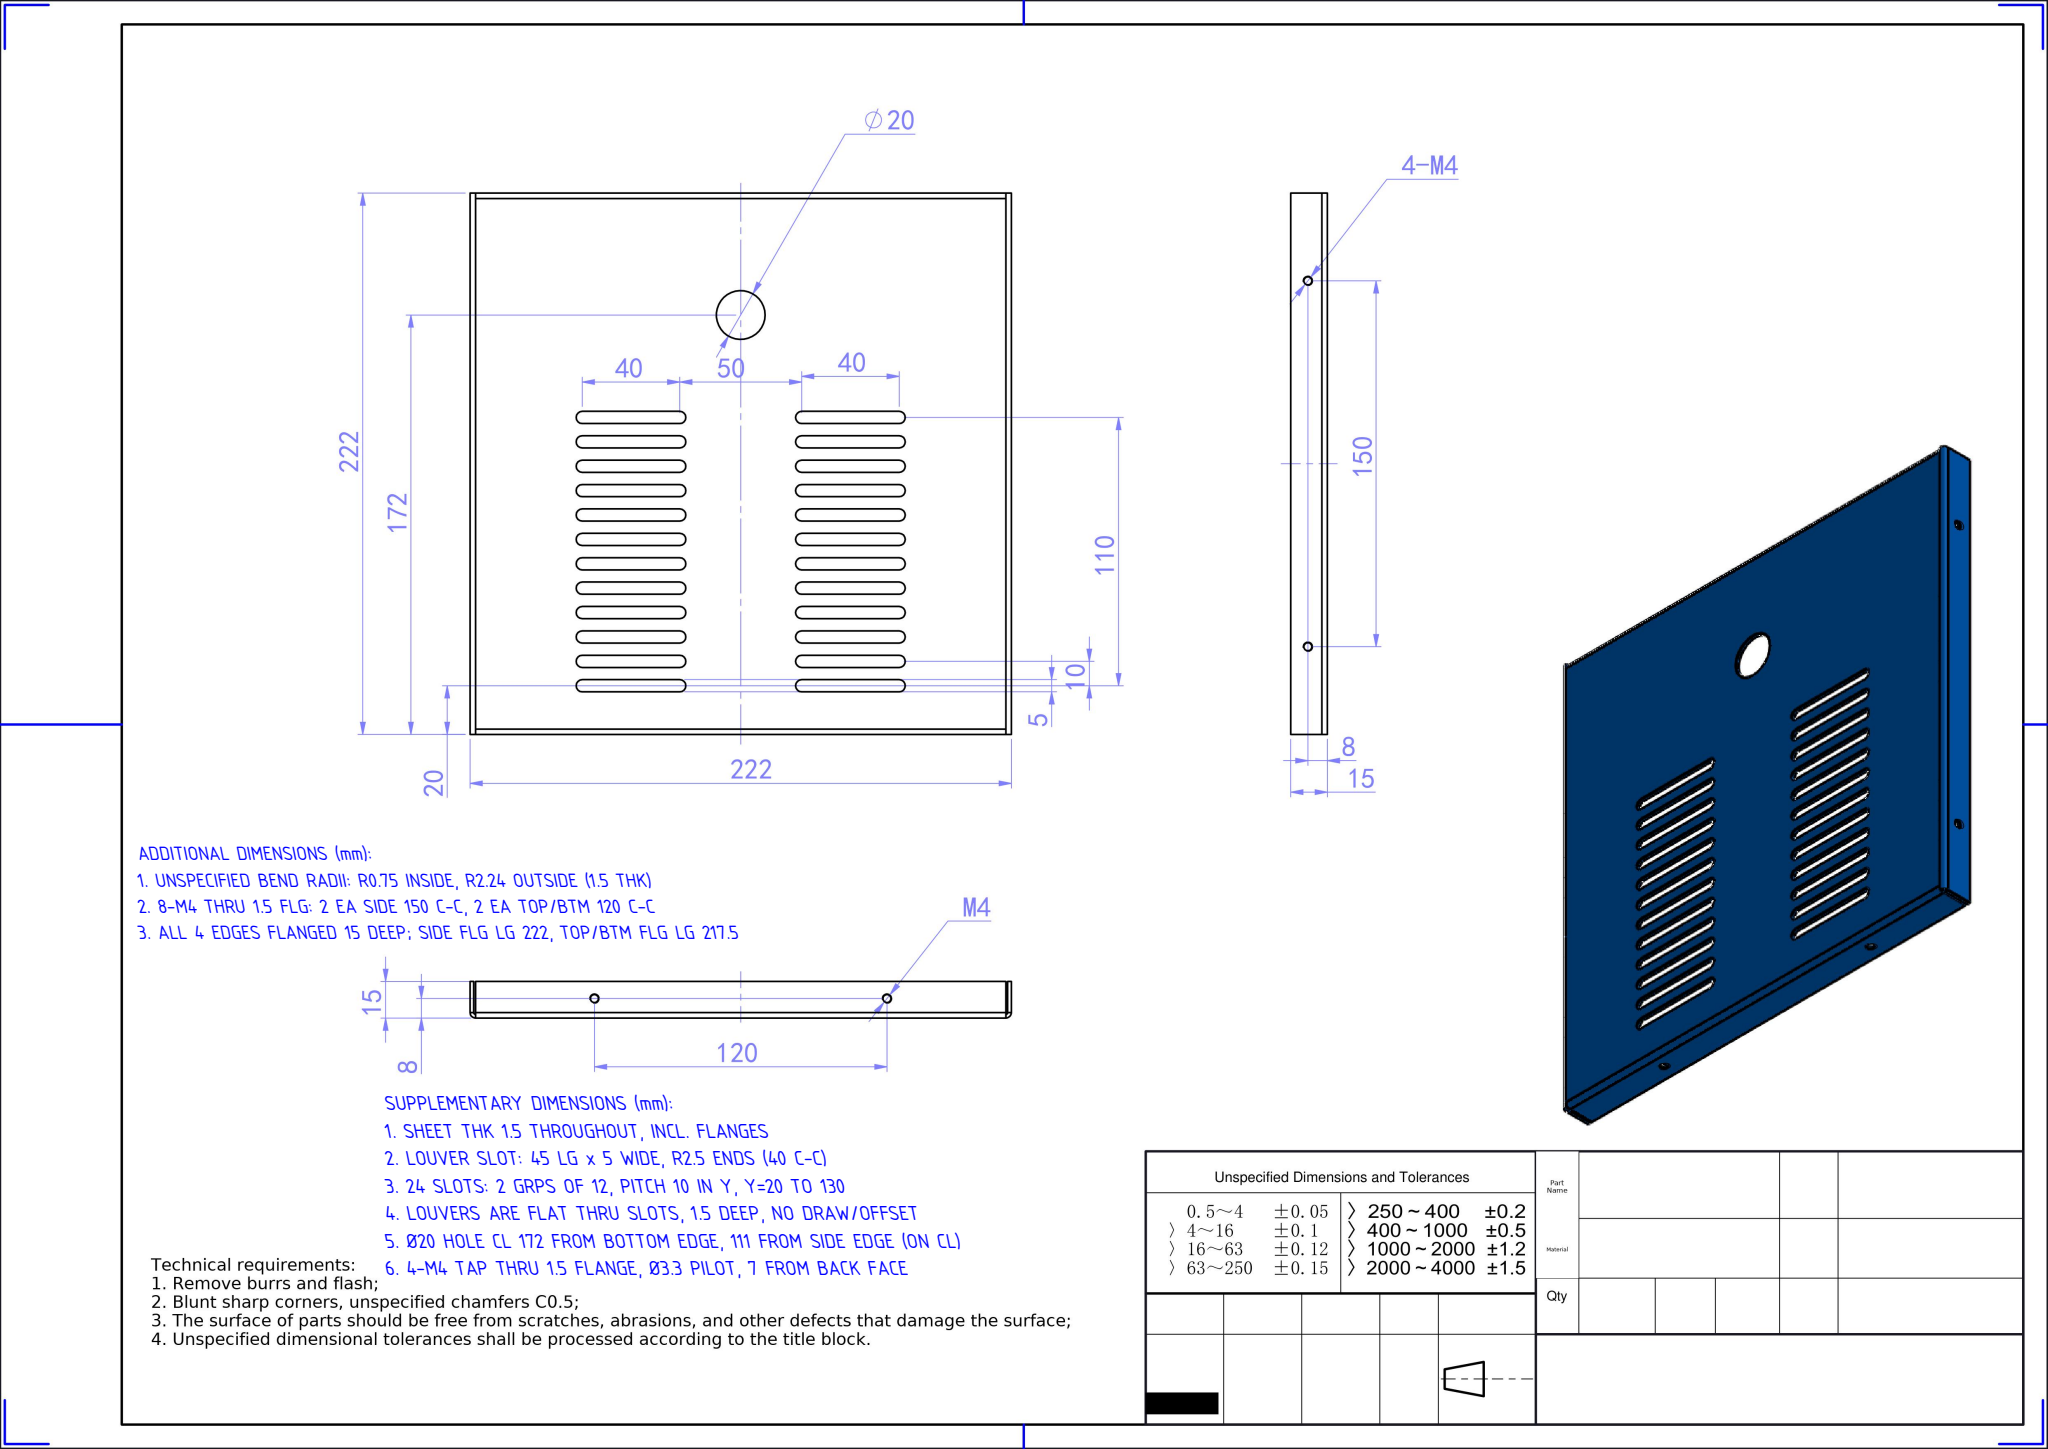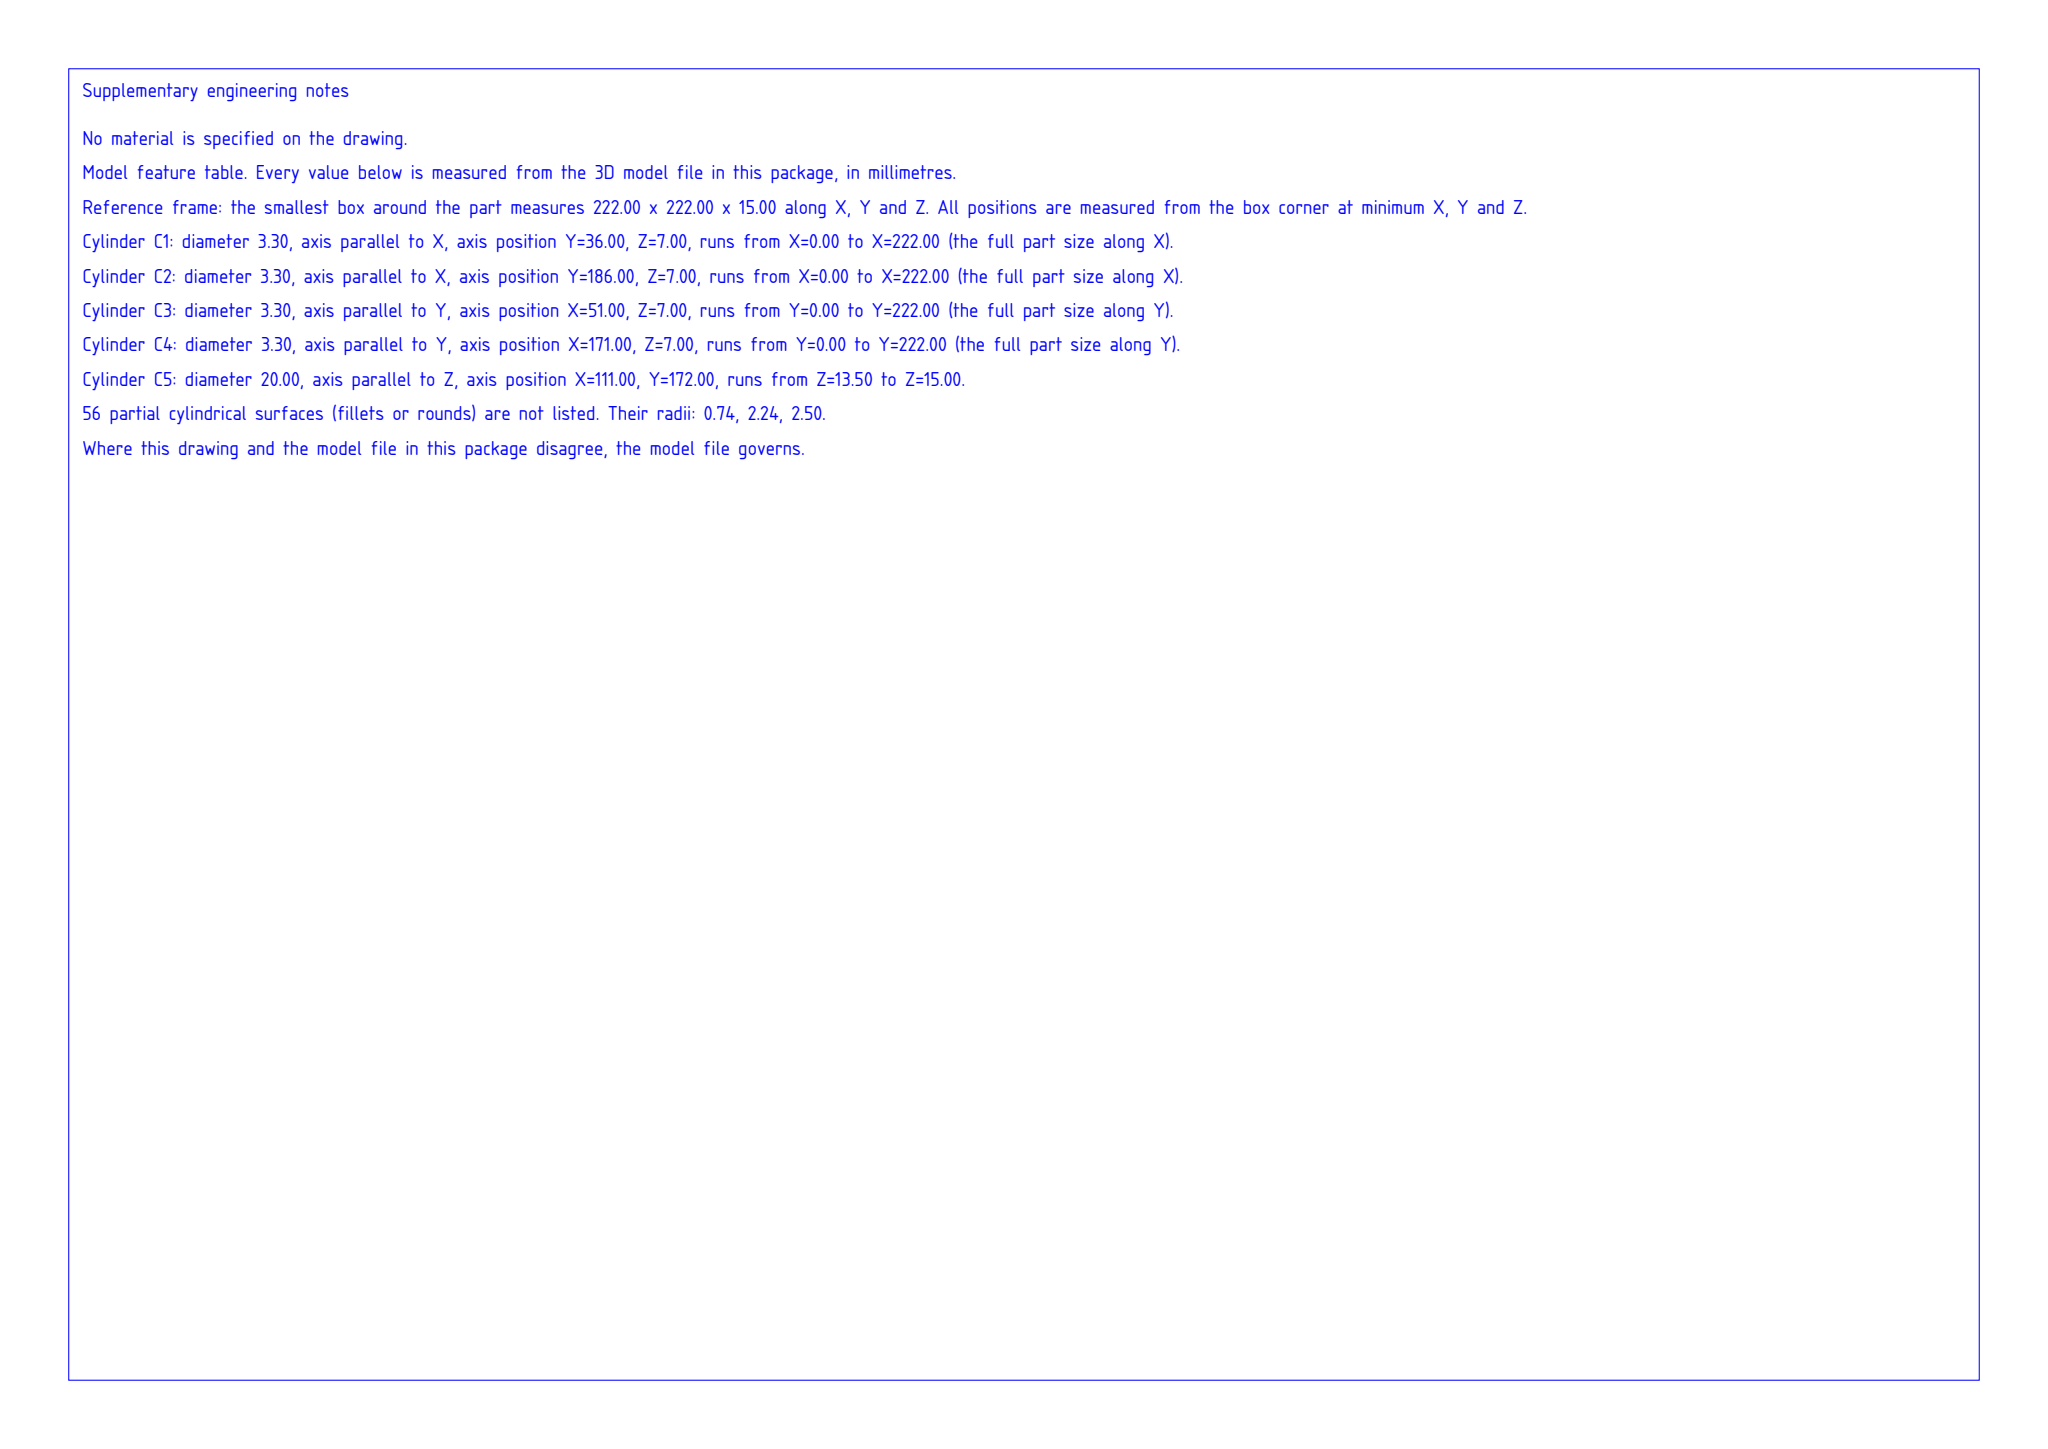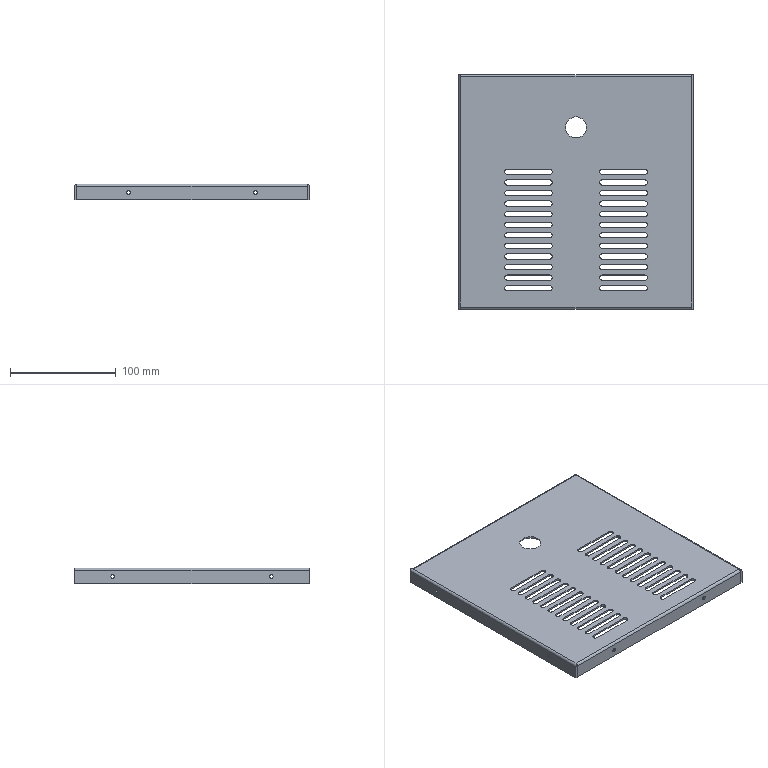Part | SolidWorks | mm | 1 solid | 180 faces | box 222 x 222 x 15 mm | volume 82405 mm3 | cylinder 98 | plane 82 | commonest cylinder face diameters 5 x72 3.3 x16 4.473 x4 1.473 x4 20 x2